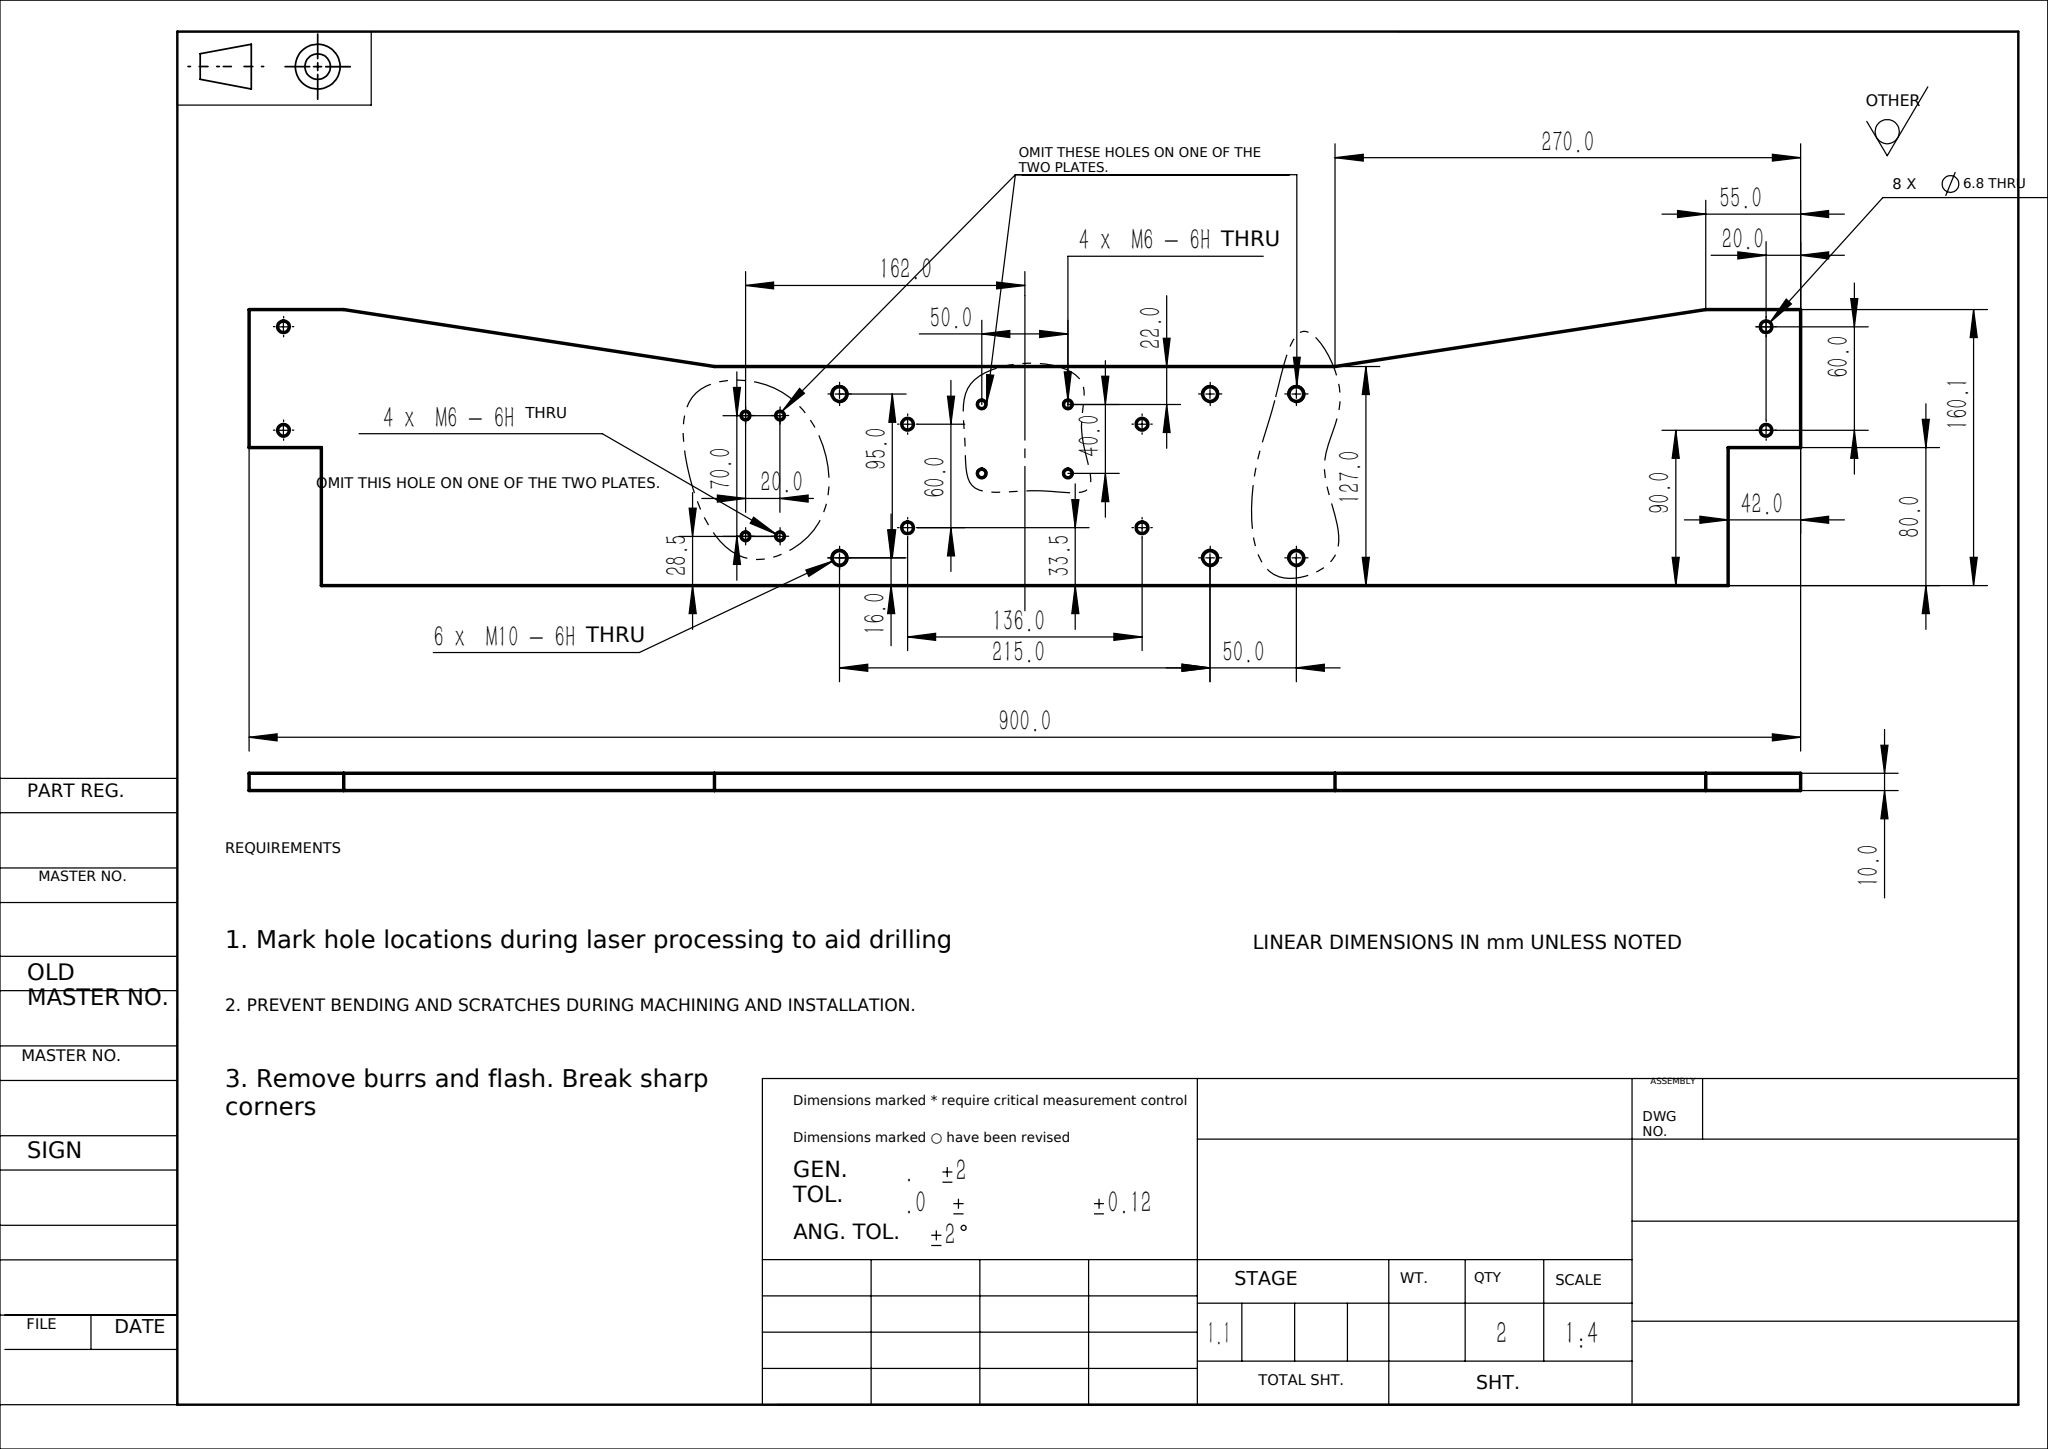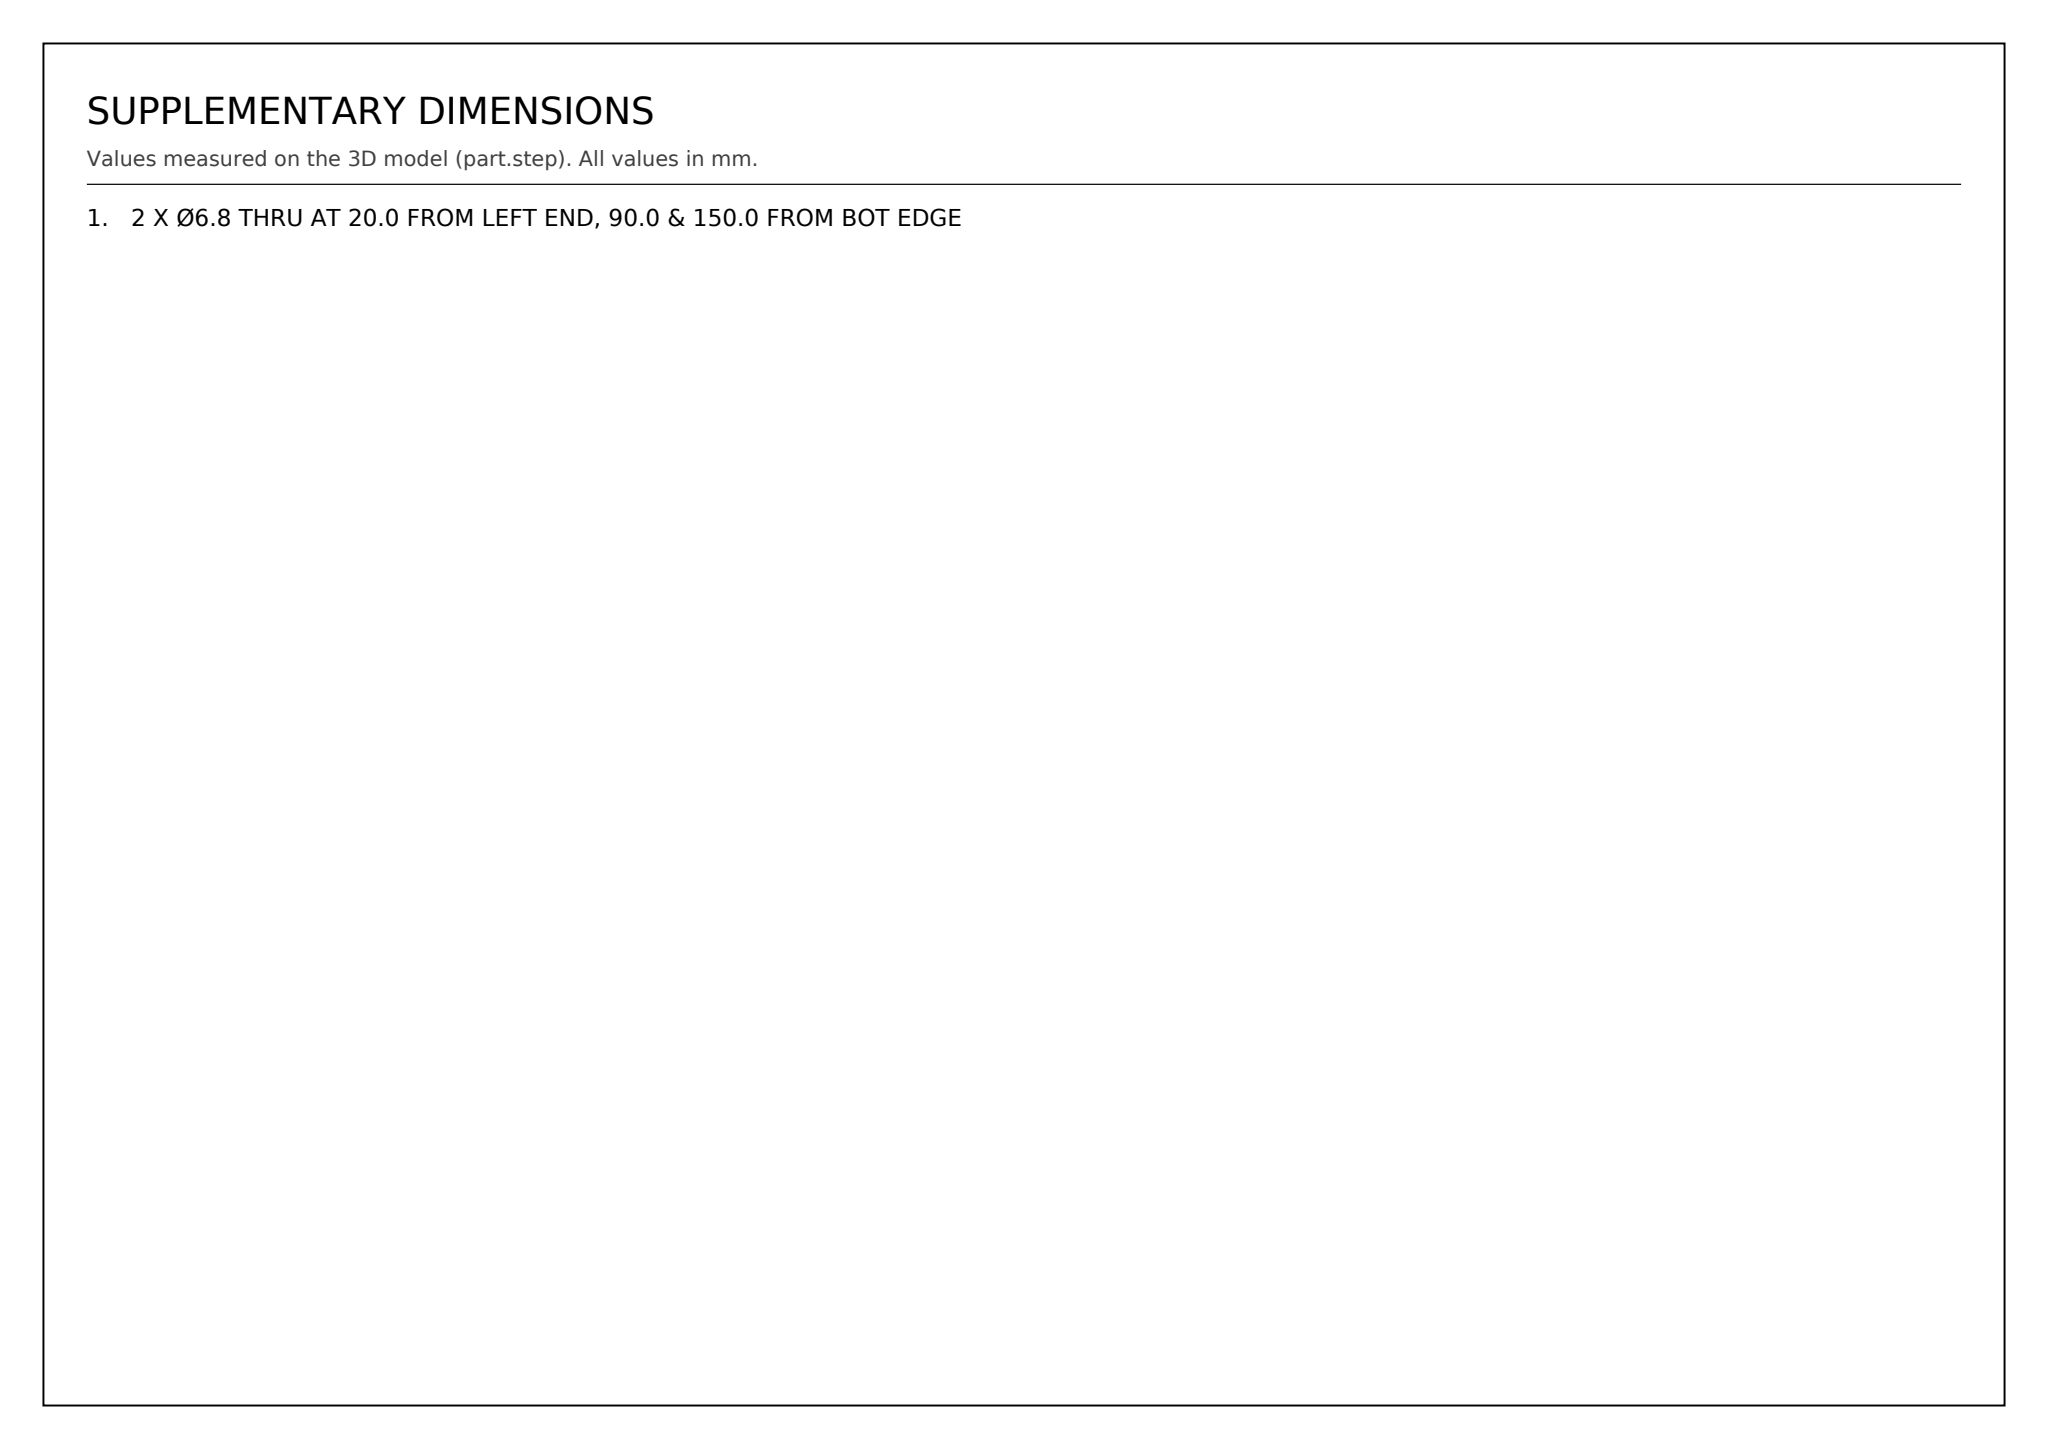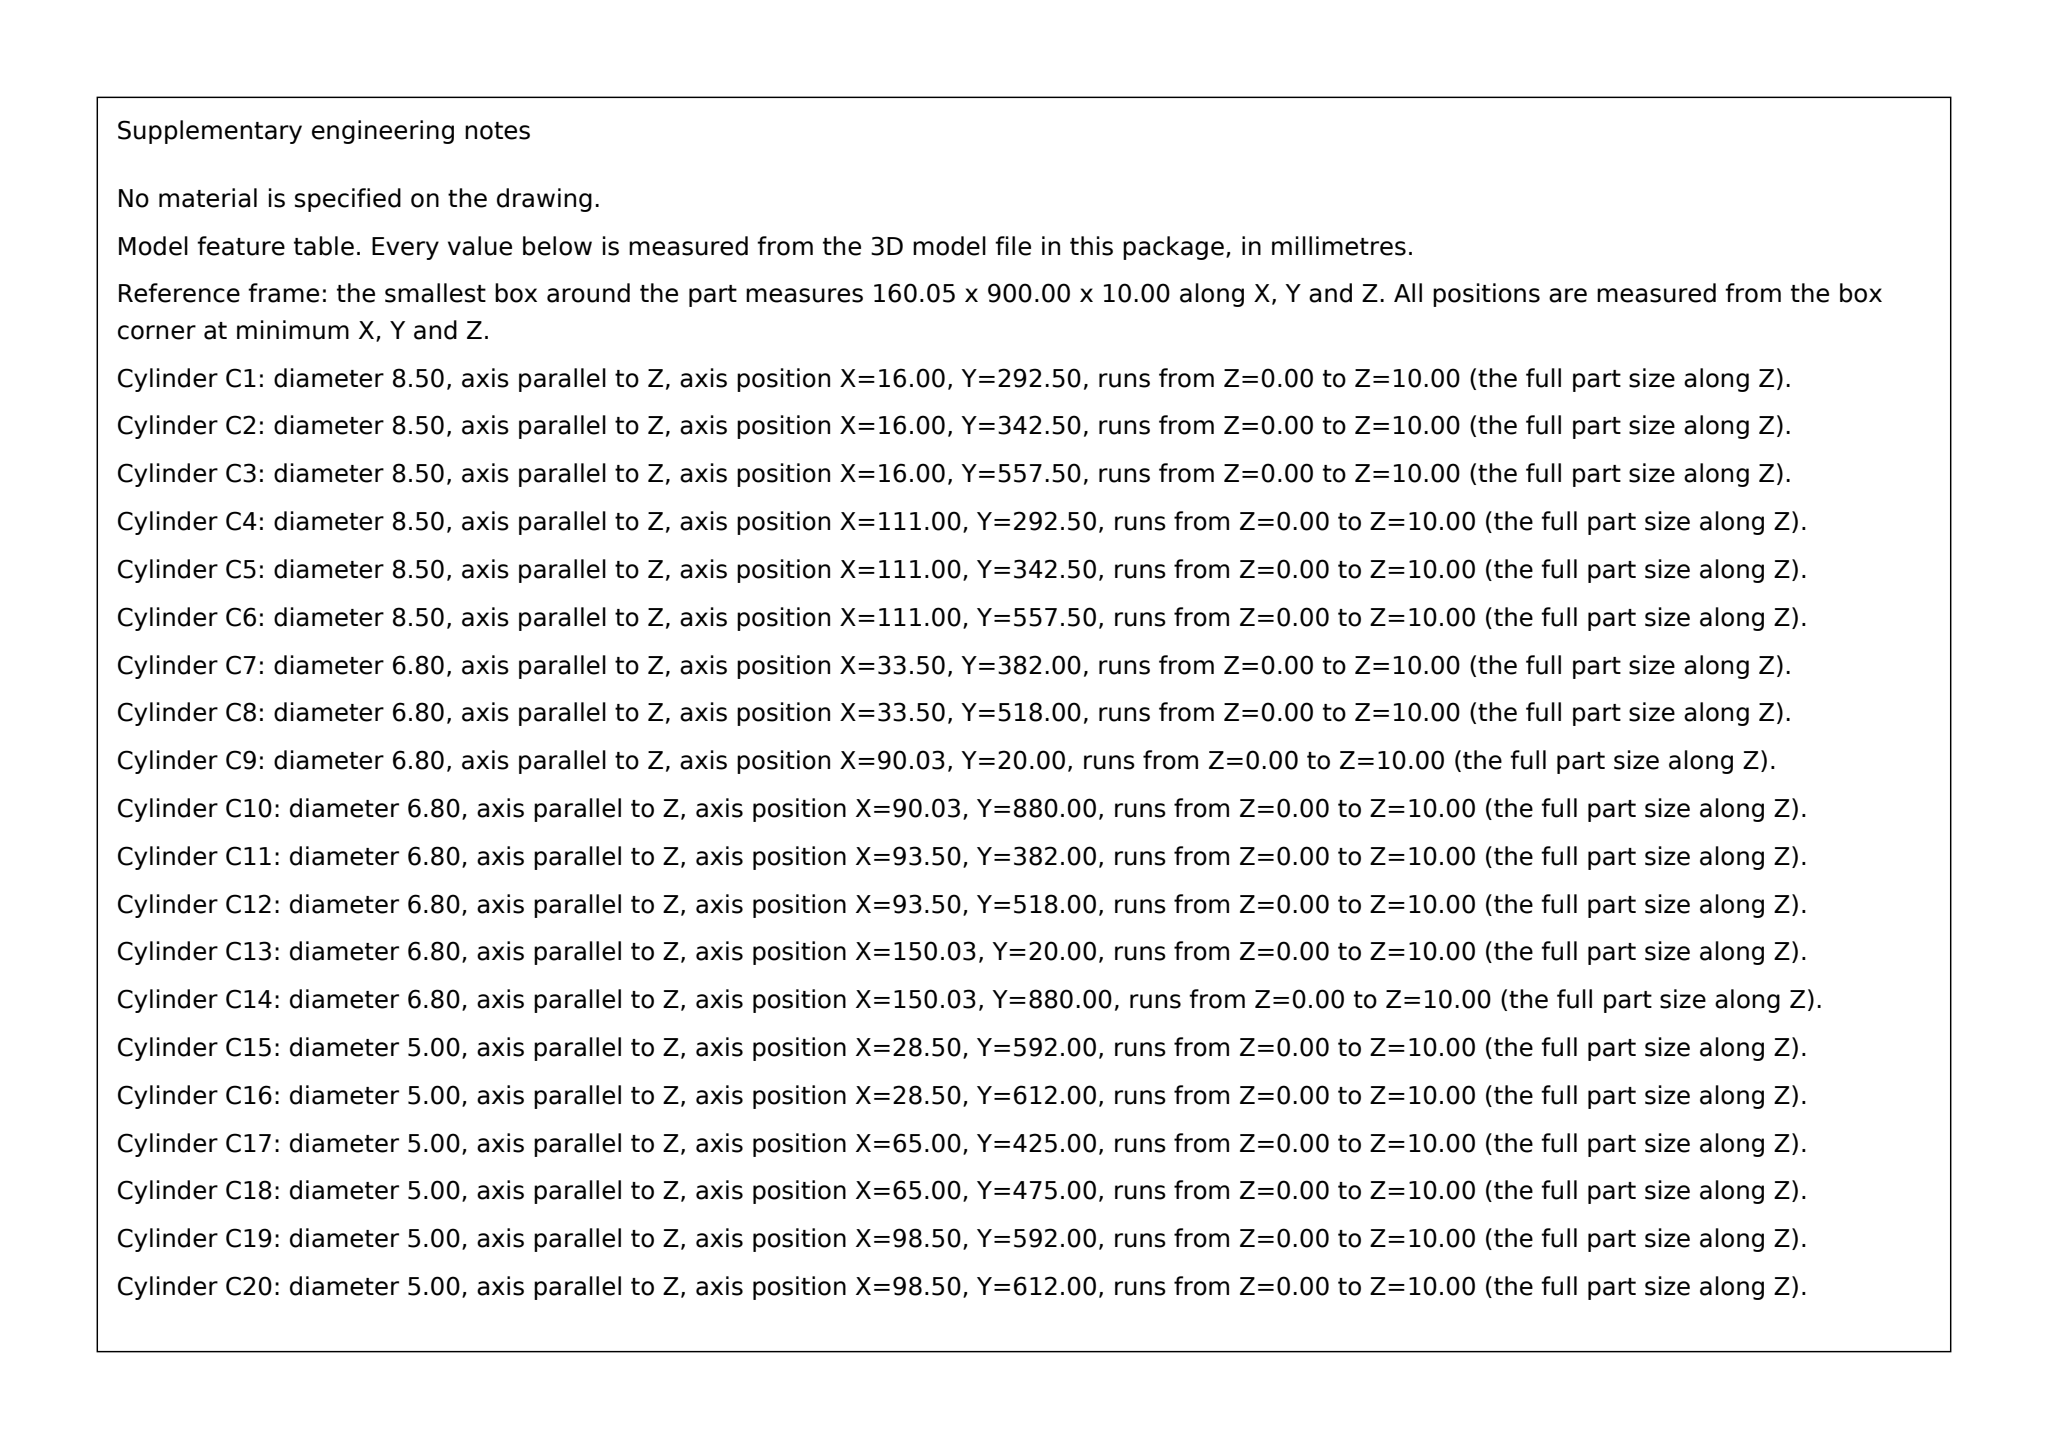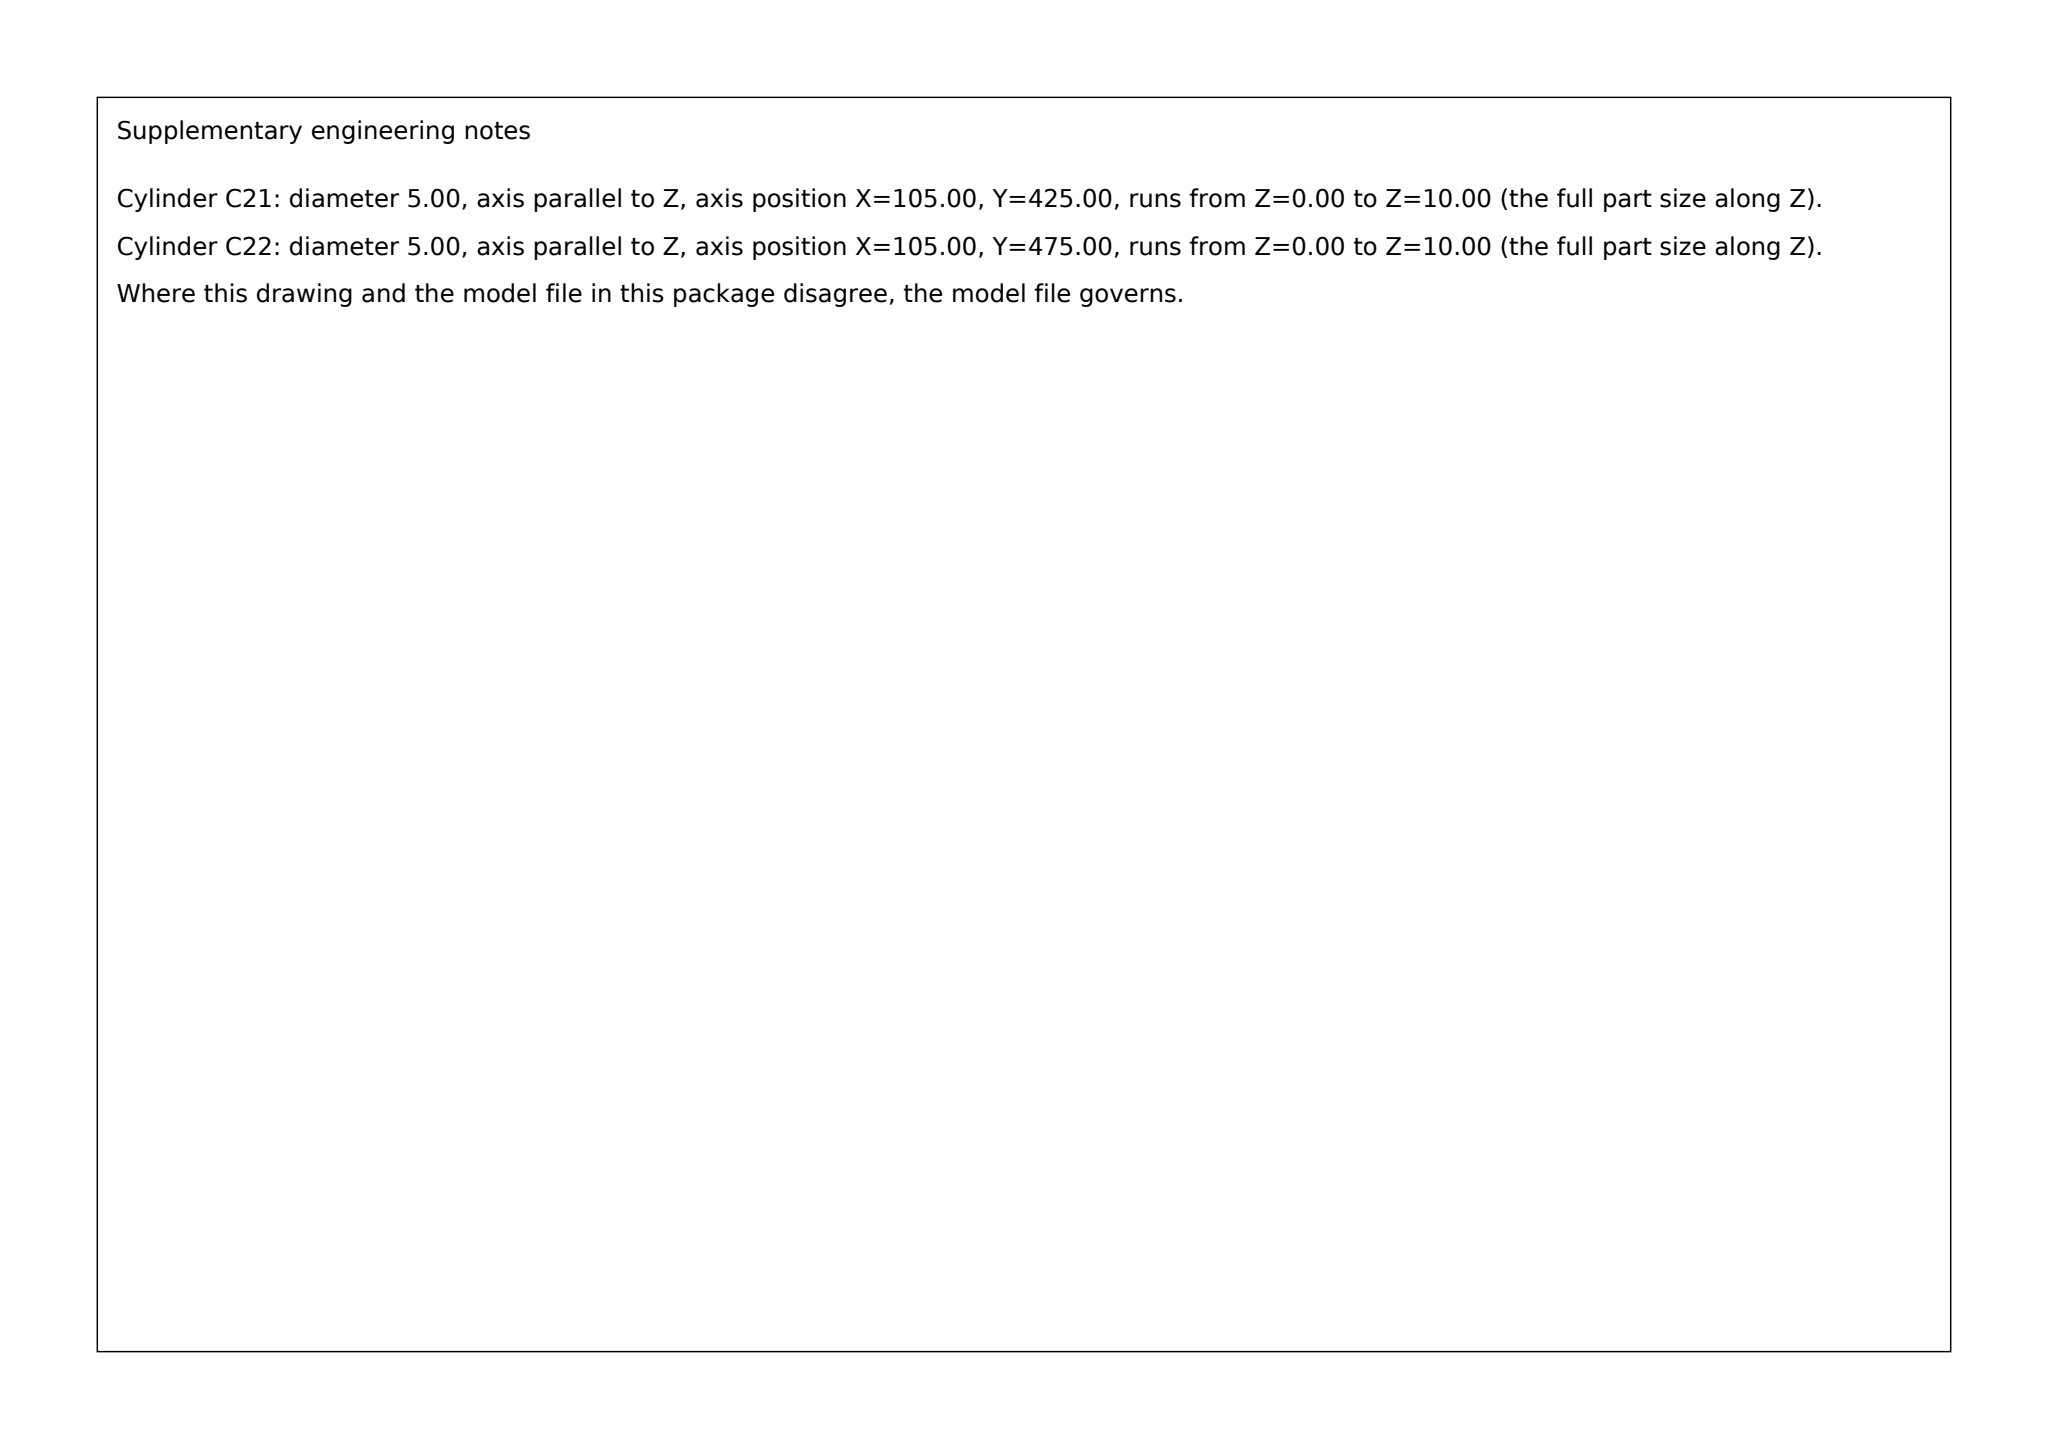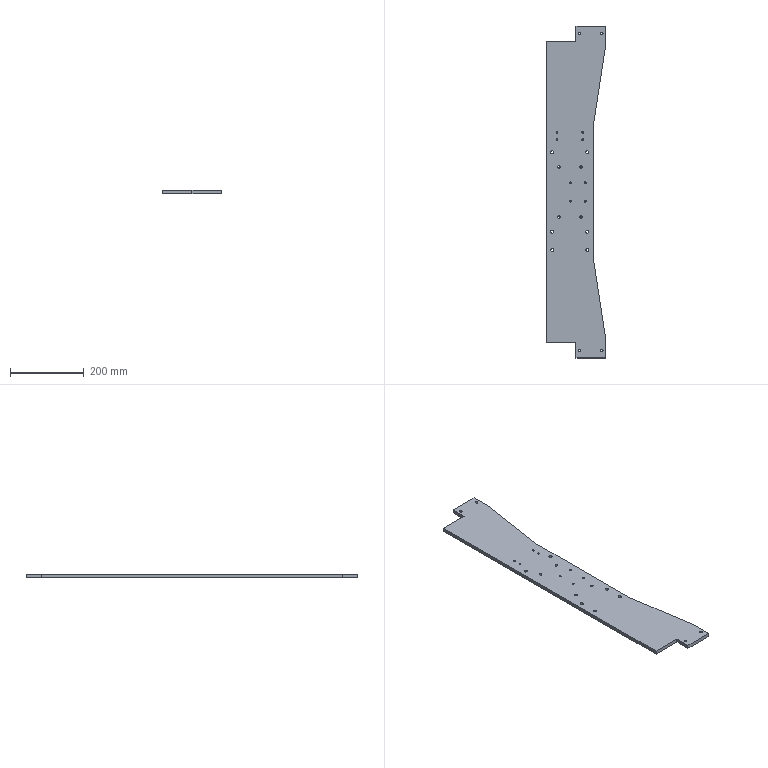Part | SolidWorks | mm | 1 solid | 58 faces | box 160.05 x 900 x 10 mm | volume 1175339 mm3 | cylinder 44 | plane 14 | commonest cylinder face diameters 5 x16 6.8 x16 8.5 x12
Drawing notes:
2 X Ø6.8 THRU AT 20.0 FROM LEFT END, 90.0 & 150.0 FROM BOT EDGE | from the solid: Cyl Ø6.8 z-axis at [90.03,880] and [150.03,880]; left end y=900, bottom edge x=0
build123d program:
from build123d import *

# Parameters (mm, degrees)
BOSS_EXTRUDE1_DEPTH        = 10
F_6_8_6_8_DIAMETER_HOLE1_D = 6.8
M10_TAPPED_HOLE1_D         = 8.5
M6_TAPPED_HOLE1_D          = 5
M6_TAPPED_HOLE2_D          = 5


with BuildPart() as part:
    # Sketch1 → Boss-Extrude1 (new body)
    with BuildSketch(Plane.XY):
        Polygon((-7912.031, -1020.325), (-7878.979, -1235.325), (-7878.979, -1290.325), (-7912.031, -1290.325), (-7959.031, -1290.325), (-7959.031, -1248.325), (-8039.031, -1248.325), (-8039.031, -432.325), (-7959.031, -432.325), (-7959.031, -390.325), (-7912.031, -390.325), (-7878.979, -390.325), (-7878.979, -445.325), (-7912.031, -660.325), align=None)
    extrude(amount=BOSS_EXTRUDE1_DEPTH)

    # 6.8 _6.8_ Diameter Hole1 (through all)
    with Locations(Plane.XY.offset(10)):
        with Locations((-7889.005, -1270.325), (-7949.005, -1270.325), (-8005.531, -908.325), (-7949.005, -410.325), (-7889.005, -410.325), (-8005.531, -772.325), (-7945.531, -772.325), (-7945.531, -908.325)):
            Hole(F_6_8_6_8_DIAMETER_HOLE1_D / 2)

    # M10 Tapped Hole1 (through all)
    with Locations(Plane.XY.offset(10)):
        with Locations((-8023.031, -732.825), (-7928.031, -732.825), (-7928.031, -947.825), (-8023.031, -947.825), (-8023.031, -997.825), (-7928.031, -997.825)):
            Hole(M10_TAPPED_HOLE1_D / 2)

    # M6 Tapped Hole1 (through all)
    with Locations(Plane.XY.offset(10)):
        with Locations((-8010.531, -698.325), (-8010.531, -678.325), (-7940.531, -698.325), (-7940.531, -678.325)):
            Hole(M6_TAPPED_HOLE1_D / 2)

    # M6 Tapped Hole2 (through all)
    with Locations(Plane.XY.offset(10)):
        with Locations((-7934.031, -865.325), (-7934.031, -815.325), (-7974.031, -815.325), (-7974.031, -865.325)):
            Hole(M6_TAPPED_HOLE2_D / 2)


solid = part.part